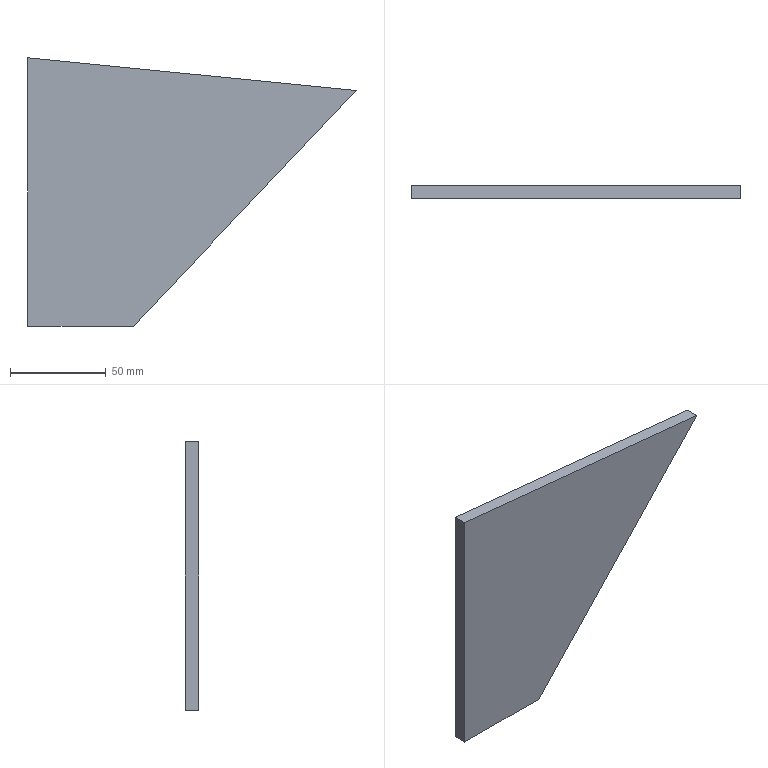Component | NX | TRIANGLE2 | 1 solid | 6 faces | box 171.17 x 7 x 140 mm | volume 107534 mm3 | plane 6
STEP:
#1=CARTESIAN_POINT('',(0.,0.,0.));
#2=DIRECTION('',(0.,0.,1.));
#3=DIRECTION('',(1.,0.,0.));
#4=AXIS2_PLACEMENT_3D('',#1,#2,#3);
#5=CARTESIAN_POINT('',(1430.,1665.,240.032));
#6=VERTEX_POINT('',#5);
#7=CARTESIAN_POINT('',(1546.175,1665.,362.943));
#8=VERTEX_POINT('',#7);
#9=CARTESIAN_POINT('',(1430.,1665.,240.032));
#10=DIRECTION('',(0.6869,0.,0.7267));
#11=VECTOR('',#10,1.);
#12=LINE('',#9,#11);
#13=CARTESIAN_POINT('',(1430.,1658.,240.032));
#14=DIRECTION('',(-0.7267,0.,0.6869));
#15=DIRECTION('',(0.6869,0.,0.7267));
#16=AXIS2_PLACEMENT_3D('',#13,#14,#15);
#17=PLANE('',#16);
#18=CARTESIAN_POINT('',(0.,7.));
#19=DIRECTION('',(1.,0.));
#20=VECTOR('',#19,1.);
#21=LINE('',#18,#20);
#22=(GEOMETRIC_REPRESENTATION_CONTEXT(2)PARAMETRIC_REPRESENTATION_CONTEXT()REPRESENTATION_CONTEXT('',''));
#23=DEFINITIONAL_REPRESENTATION('',(#21),#22);
#24=PCURVE('',#17,#23);
#25=CARTESIAN_POINT('',(1546.175,1665.,362.943));
#26=DIRECTION('',(0.,-1.,0.));
#27=DIRECTION('',(0.,0.,-1.));
#28=AXIS2_PLACEMENT_3D('',#25,#26,#27);
#29=PLANE('',#28);
#30=CARTESIAN_POINT('',(122.911,-116.175));
#31=DIRECTION('',(-0.7267,0.6869));
#32=VECTOR('',#31,1.);
#33=LINE('',#30,#32);
#34=(GEOMETRIC_REPRESENTATION_CONTEXT(2)PARAMETRIC_REPRESENTATION_CONTEXT()REPRESENTATION_CONTEXT('',''));
#35=DEFINITIONAL_REPRESENTATION('',(#33),#34);
#36=PCURVE('',#29,#35);
#37=SURFACE_CURVE('',#12,(#24,#36),.PCURVE_S1.);
#38=EDGE_CURVE('',#6,#8,#37,.T.);
#39=ORIENTED_EDGE('',*,*,#38,.T.);
#40=CARTESIAN_POINT('',(1546.175,1658.,362.943));
#41=VERTEX_POINT('',#40);
#42=CARTESIAN_POINT('',(1546.175,1658.,362.943));
#43=DIRECTION('',(0.,1.,0.));
#44=VECTOR('',#43,1.);
#45=LINE('',#42,#44);
#46=CARTESIAN_POINT('',(169.127,0.));
#47=DIRECTION('',(0.,1.));
#48=VECTOR('',#47,1.);
#49=LINE('',#46,#48);
#50=(GEOMETRIC_REPRESENTATION_CONTEXT(2)PARAMETRIC_REPRESENTATION_CONTEXT()REPRESENTATION_CONTEXT('',''));
#51=DEFINITIONAL_REPRESENTATION('',(#49),#50);
#52=PCURVE('',#17,#51);
#53=CARTESIAN_POINT('',(1546.175,1658.,362.943));
#54=DIRECTION('',(-0.09932,0.,-0.9951));
#55=DIRECTION('',(-0.9951,0.,0.09932));
#56=AXIS2_PLACEMENT_3D('',#53,#54,#55);
#57=PLANE('',#56);
#58=CARTESIAN_POINT('',(0.,0.));
#59=DIRECTION('',(0.,1.));
#60=VECTOR('',#59,1.);
#61=LINE('',#58,#60);
#62=(GEOMETRIC_REPRESENTATION_CONTEXT(2)PARAMETRIC_REPRESENTATION_CONTEXT()REPRESENTATION_CONTEXT('',''));
#63=DEFINITIONAL_REPRESENTATION('',(#61),#62);
#64=PCURVE('',#57,#63);
#65=SURFACE_CURVE('',#45,(#52,#64),.PCURVE_S1.);
#66=EDGE_CURVE('',#41,#8,#65,.T.);
#67=ORIENTED_EDGE('',*,*,#66,.F.);
#68=CARTESIAN_POINT('',(1430.,1658.,240.032));
#69=VERTEX_POINT('',#68);
#70=CARTESIAN_POINT('',(1430.,1658.,240.032));
#71=DIRECTION('',(0.6869,0.,0.7267));
#72=VECTOR('',#71,1.);
#73=LINE('',#70,#72);
#74=CARTESIAN_POINT('',(0.,0.));
#75=DIRECTION('',(1.,0.));
#76=VECTOR('',#75,1.);
#77=LINE('',#74,#76);
#78=(GEOMETRIC_REPRESENTATION_CONTEXT(2)PARAMETRIC_REPRESENTATION_CONTEXT()REPRESENTATION_CONTEXT('',''));
#79=DEFINITIONAL_REPRESENTATION('',(#77),#78);
#80=PCURVE('',#17,#79);
#81=CARTESIAN_POINT('',(1546.175,1658.,362.943));
#82=DIRECTION('',(0.,-1.,0.));
#83=DIRECTION('',(0.,0.,-1.));
#84=AXIS2_PLACEMENT_3D('',#81,#82,#83);
#85=PLANE('',#84);
#86=CARTESIAN_POINT('',(122.911,-116.175));
#87=DIRECTION('',(-0.7267,0.6869));
#88=VECTOR('',#87,1.);
#89=LINE('',#86,#88);
#90=(GEOMETRIC_REPRESENTATION_CONTEXT(2)PARAMETRIC_REPRESENTATION_CONTEXT()REPRESENTATION_CONTEXT('',''));
#91=DEFINITIONAL_REPRESENTATION('',(#89),#90);
#92=PCURVE('',#85,#91);
#93=SURFACE_CURVE('',#73,(#80,#92),.PCURVE_S1.);
#94=EDGE_CURVE('',#69,#41,#93,.T.);
#95=ORIENTED_EDGE('',*,*,#94,.F.);
#96=CARTESIAN_POINT('',(1430.,1658.,240.032));
#97=DIRECTION('',(0.,1.,0.));
#98=VECTOR('',#97,1.);
#99=LINE('',#96,#98);
#100=CARTESIAN_POINT('',(0.,0.));
#101=DIRECTION('',(0.,1.));
#102=VECTOR('',#101,1.);
#103=LINE('',#100,#102);
#104=(GEOMETRIC_REPRESENTATION_CONTEXT(2)PARAMETRIC_REPRESENTATION_CONTEXT()REPRESENTATION_CONTEXT('',''));
#105=DEFINITIONAL_REPRESENTATION('',(#103),#104);
#106=PCURVE('',#17,#105);
#107=CARTESIAN_POINT('',(1375.,1658.,240.032));
#108=DIRECTION('',(0.,0.,1.));
#109=DIRECTION('',(1.,0.,-0.));
#110=AXIS2_PLACEMENT_3D('',#107,#108,#109);
#111=PLANE('',#110);
#112=CARTESIAN_POINT('',(55.,0.));
#113=DIRECTION('',(0.,1.));
#114=VECTOR('',#113,1.);
#115=LINE('',#112,#114);
#116=(GEOMETRIC_REPRESENTATION_CONTEXT(2)PARAMETRIC_REPRESENTATION_CONTEXT()REPRESENTATION_CONTEXT('',''));
#117=DEFINITIONAL_REPRESENTATION('',(#115),#116);
#118=PCURVE('',#111,#117);
#119=SURFACE_CURVE('',#99,(#106,#118),.PCURVE_S1.);
#120=EDGE_CURVE('',#69,#6,#119,.T.);
#121=ORIENTED_EDGE('',*,*,#120,.T.);
#122=EDGE_LOOP('',(#39,#67,#95,#121));
#123=FACE_BOUND('',#122,.T.);
#124=ADVANCED_FACE('',(#123),#17,.F.);
#125=CARTESIAN_POINT('',(1375.,1665.,380.029));
#126=VERTEX_POINT('',#125);
#127=CARTESIAN_POINT('',(1546.175,1665.,362.943));
#128=DIRECTION('',(-0.9951,0.,0.09932));
#129=VECTOR('',#128,1.);
#130=LINE('',#127,#129);
#131=CARTESIAN_POINT('',(0.,7.));
#132=DIRECTION('',(1.,0.));
#133=VECTOR('',#132,1.);
#134=LINE('',#131,#133);
#135=(GEOMETRIC_REPRESENTATION_CONTEXT(2)PARAMETRIC_REPRESENTATION_CONTEXT()REPRESENTATION_CONTEXT('',''));
#136=DEFINITIONAL_REPRESENTATION('',(#134),#135);
#137=PCURVE('',#57,#136);
#138=CARTESIAN_POINT('',(0.,0.));
#139=DIRECTION('',(-0.09932,-0.9951));
#140=VECTOR('',#139,1.);
#141=LINE('',#138,#140);
#142=(GEOMETRIC_REPRESENTATION_CONTEXT(2)PARAMETRIC_REPRESENTATION_CONTEXT()REPRESENTATION_CONTEXT('',''));
#143=DEFINITIONAL_REPRESENTATION('',(#141),#142);
#144=PCURVE('',#29,#143);
#145=SURFACE_CURVE('',#130,(#137,#144),.PCURVE_S1.);
#146=EDGE_CURVE('',#8,#126,#145,.T.);
#147=ORIENTED_EDGE('',*,*,#146,.T.);
#148=CARTESIAN_POINT('',(1375.,1658.,380.029));
#149=VERTEX_POINT('',#148);
#150=CARTESIAN_POINT('',(1375.,1658.,380.029));
#151=DIRECTION('',(0.,1.,0.));
#152=VECTOR('',#151,1.);
#153=LINE('',#150,#152);
#154=CARTESIAN_POINT('',(172.025,0.));
#155=DIRECTION('',(0.,1.));
#156=VECTOR('',#155,1.);
#157=LINE('',#154,#156);
#158=(GEOMETRIC_REPRESENTATION_CONTEXT(2)PARAMETRIC_REPRESENTATION_CONTEXT()REPRESENTATION_CONTEXT('',''));
#159=DEFINITIONAL_REPRESENTATION('',(#157),#158);
#160=PCURVE('',#57,#159);
#161=CARTESIAN_POINT('',(1375.,1658.,380.029));
#162=DIRECTION('',(1.,0.,0.));
#163=DIRECTION('',(0.,0.,-1.));
#164=AXIS2_PLACEMENT_3D('',#161,#162,#163);
#165=PLANE('',#164);
#166=CARTESIAN_POINT('',(0.,0.));
#167=DIRECTION('',(0.,1.));
#168=VECTOR('',#167,1.);
#169=LINE('',#166,#168);
#170=(GEOMETRIC_REPRESENTATION_CONTEXT(2)PARAMETRIC_REPRESENTATION_CONTEXT()REPRESENTATION_CONTEXT('',''));
#171=DEFINITIONAL_REPRESENTATION('',(#169),#170);
#172=PCURVE('',#165,#171);
#173=SURFACE_CURVE('',#153,(#160,#172),.PCURVE_S1.);
#174=EDGE_CURVE('',#149,#126,#173,.T.);
#175=ORIENTED_EDGE('',*,*,#174,.F.);
#176=CARTESIAN_POINT('',(1546.175,1658.,362.943));
#177=DIRECTION('',(-0.9951,0.,0.09932));
#178=VECTOR('',#177,1.);
#179=LINE('',#176,#178);
#180=CARTESIAN_POINT('',(0.,0.));
#181=DIRECTION('',(1.,0.));
#182=VECTOR('',#181,1.);
#183=LINE('',#180,#182);
#184=(GEOMETRIC_REPRESENTATION_CONTEXT(2)PARAMETRIC_REPRESENTATION_CONTEXT()REPRESENTATION_CONTEXT('',''));
#185=DEFINITIONAL_REPRESENTATION('',(#183),#184);
#186=PCURVE('',#57,#185);
#187=CARTESIAN_POINT('',(0.,0.));
#188=DIRECTION('',(-0.09932,-0.9951));
#189=VECTOR('',#188,1.);
#190=LINE('',#187,#189);
#191=(GEOMETRIC_REPRESENTATION_CONTEXT(2)PARAMETRIC_REPRESENTATION_CONTEXT()REPRESENTATION_CONTEXT('',''));
#192=DEFINITIONAL_REPRESENTATION('',(#190),#191);
#193=PCURVE('',#85,#192);
#194=SURFACE_CURVE('',#179,(#186,#193),.PCURVE_S1.);
#195=EDGE_CURVE('',#41,#149,#194,.T.);
#196=ORIENTED_EDGE('',*,*,#195,.F.);
#197=ORIENTED_EDGE('',*,*,#66,.T.);
#198=EDGE_LOOP('',(#147,#175,#196,#197));
#199=FACE_BOUND('',#198,.T.);
#200=ADVANCED_FACE('',(#199),#57,.F.);
#201=CARTESIAN_POINT('',(1375.,1665.,240.032));
#202=VERTEX_POINT('',#201);
#203=CARTESIAN_POINT('',(1375.,1665.,380.029));
#204=DIRECTION('',(0.,0.,-1.));
#205=VECTOR('',#204,1.);
#206=LINE('',#203,#205);
#207=CARTESIAN_POINT('',(0.,7.));
#208=DIRECTION('',(1.,0.));
#209=VECTOR('',#208,1.);
#210=LINE('',#207,#209);
#211=(GEOMETRIC_REPRESENTATION_CONTEXT(2)PARAMETRIC_REPRESENTATION_CONTEXT()REPRESENTATION_CONTEXT('',''));
#212=DEFINITIONAL_REPRESENTATION('',(#210),#211);
#213=PCURVE('',#165,#212);
#214=CARTESIAN_POINT('',(-17.086,-171.175));
#215=DIRECTION('',(1.,0.));
#216=VECTOR('',#215,1.);
#217=LINE('',#214,#216);
#218=(GEOMETRIC_REPRESENTATION_CONTEXT(2)PARAMETRIC_REPRESENTATION_CONTEXT()REPRESENTATION_CONTEXT('',''));
#219=DEFINITIONAL_REPRESENTATION('',(#217),#218);
#220=PCURVE('',#29,#219);
#221=SURFACE_CURVE('',#206,(#213,#220),.PCURVE_S1.);
#222=EDGE_CURVE('',#126,#202,#221,.T.);
#223=ORIENTED_EDGE('',*,*,#222,.T.);
#224=CARTESIAN_POINT('',(1375.,1658.,240.032));
#225=VERTEX_POINT('',#224);
#226=CARTESIAN_POINT('',(1375.,1658.,240.032));
#227=DIRECTION('',(0.,1.,0.));
#228=VECTOR('',#227,1.);
#229=LINE('',#226,#228);
#230=CARTESIAN_POINT('',(139.997,0.));
#231=DIRECTION('',(0.,1.));
#232=VECTOR('',#231,1.);
#233=LINE('',#230,#232);
#234=(GEOMETRIC_REPRESENTATION_CONTEXT(2)PARAMETRIC_REPRESENTATION_CONTEXT()REPRESENTATION_CONTEXT('',''));
#235=DEFINITIONAL_REPRESENTATION('',(#233),#234);
#236=PCURVE('',#165,#235);
#237=CARTESIAN_POINT('',(0.,0.));
#238=DIRECTION('',(0.,1.));
#239=VECTOR('',#238,1.);
#240=LINE('',#237,#239);
#241=(GEOMETRIC_REPRESENTATION_CONTEXT(2)PARAMETRIC_REPRESENTATION_CONTEXT()REPRESENTATION_CONTEXT('',''));
#242=DEFINITIONAL_REPRESENTATION('',(#240),#241);
#243=PCURVE('',#111,#242);
#244=SURFACE_CURVE('',#229,(#236,#243),.PCURVE_S1.);
#245=EDGE_CURVE('',#225,#202,#244,.T.);
#246=ORIENTED_EDGE('',*,*,#245,.F.);
#247=CARTESIAN_POINT('',(1375.,1658.,380.029));
#248=DIRECTION('',(0.,0.,-1.));
#249=VECTOR('',#248,1.);
#250=LINE('',#247,#249);
#251=CARTESIAN_POINT('',(0.,0.));
#252=DIRECTION('',(1.,0.));
#253=VECTOR('',#252,1.);
#254=LINE('',#251,#253);
#255=(GEOMETRIC_REPRESENTATION_CONTEXT(2)PARAMETRIC_REPRESENTATION_CONTEXT()REPRESENTATION_CONTEXT('',''));
#256=DEFINITIONAL_REPRESENTATION('',(#254),#255);
#257=PCURVE('',#165,#256);
#258=CARTESIAN_POINT('',(-17.086,-171.175));
#259=DIRECTION('',(1.,0.));
#260=VECTOR('',#259,1.);
#261=LINE('',#258,#260);
#262=(GEOMETRIC_REPRESENTATION_CONTEXT(2)PARAMETRIC_REPRESENTATION_CONTEXT()REPRESENTATION_CONTEXT('',''));
#263=DEFINITIONAL_REPRESENTATION('',(#261),#262);
#264=PCURVE('',#85,#263);
#265=SURFACE_CURVE('',#250,(#257,#264),.PCURVE_S1.);
#266=EDGE_CURVE('',#149,#225,#265,.T.);
#267=ORIENTED_EDGE('',*,*,#266,.F.);
#268=ORIENTED_EDGE('',*,*,#174,.T.);
#269=EDGE_LOOP('',(#223,#246,#267,#268));
#270=FACE_BOUND('',#269,.T.);
#271=ADVANCED_FACE('',(#270),#165,.F.);
#272=CARTESIAN_POINT('',(1375.,1665.,240.032));
#273=DIRECTION('',(1.,0.,-0.));
#274=VECTOR('',#273,1.);
#275=LINE('',#272,#274);
#276=CARTESIAN_POINT('',(0.,7.));
#277=DIRECTION('',(1.,0.));
#278=VECTOR('',#277,1.);
#279=LINE('',#276,#278);
#280=(GEOMETRIC_REPRESENTATION_CONTEXT(2)PARAMETRIC_REPRESENTATION_CONTEXT()REPRESENTATION_CONTEXT('',''));
#281=DEFINITIONAL_REPRESENTATION('',(#279),#280);
#282=PCURVE('',#111,#281);
#283=CARTESIAN_POINT('',(122.911,-171.175));
#284=DIRECTION('',(0.,1.));
#285=VECTOR('',#284,1.);
#286=LINE('',#283,#285);
#287=(GEOMETRIC_REPRESENTATION_CONTEXT(2)PARAMETRIC_REPRESENTATION_CONTEXT()REPRESENTATION_CONTEXT('',''));
#288=DEFINITIONAL_REPRESENTATION('',(#286),#287);
#289=PCURVE('',#29,#288);
#290=SURFACE_CURVE('',#275,(#282,#289),.PCURVE_S1.);
#291=EDGE_CURVE('',#202,#6,#290,.T.);
#292=ORIENTED_EDGE('',*,*,#291,.T.);
#293=ORIENTED_EDGE('',*,*,#120,.F.);
#294=CARTESIAN_POINT('',(1375.,1658.,240.032));
#295=DIRECTION('',(1.,0.,-0.));
#296=VECTOR('',#295,1.);
#297=LINE('',#294,#296);
#298=CARTESIAN_POINT('',(0.,0.));
#299=DIRECTION('',(1.,0.));
#300=VECTOR('',#299,1.);
#301=LINE('',#298,#300);
#302=(GEOMETRIC_REPRESENTATION_CONTEXT(2)PARAMETRIC_REPRESENTATION_CONTEXT()REPRESENTATION_CONTEXT('',''));
#303=DEFINITIONAL_REPRESENTATION('',(#301),#302);
#304=PCURVE('',#111,#303);
#305=CARTESIAN_POINT('',(122.911,-171.175));
#306=DIRECTION('',(0.,1.));
#307=VECTOR('',#306,1.);
#308=LINE('',#305,#307);
#309=(GEOMETRIC_REPRESENTATION_CONTEXT(2)PARAMETRIC_REPRESENTATION_CONTEXT()REPRESENTATION_CONTEXT('',''));
#310=DEFINITIONAL_REPRESENTATION('',(#308),#309);
#311=PCURVE('',#85,#310);
#312=SURFACE_CURVE('',#297,(#304,#311),.PCURVE_S1.);
#313=EDGE_CURVE('',#225,#69,#312,.T.);
#314=ORIENTED_EDGE('',*,*,#313,.F.);
#315=ORIENTED_EDGE('',*,*,#245,.T.);
#316=EDGE_LOOP('',(#292,#293,#314,#315));
#317=FACE_BOUND('',#316,.T.);
#318=ADVANCED_FACE('',(#317),#111,.F.);
#319=ORIENTED_EDGE('',*,*,#94,.T.);
#320=ORIENTED_EDGE('',*,*,#195,.T.);
#321=ORIENTED_EDGE('',*,*,#266,.T.);
#322=ORIENTED_EDGE('',*,*,#313,.T.);
#323=EDGE_LOOP('',(#319,#320,#321,#322));
#324=FACE_BOUND('',#323,.T.);
#325=ADVANCED_FACE('',(#324),#85,.T.);
#326=ORIENTED_EDGE('',*,*,#38,.F.);
#327=ORIENTED_EDGE('',*,*,#291,.F.);
#328=ORIENTED_EDGE('',*,*,#222,.F.);
#329=ORIENTED_EDGE('',*,*,#146,.F.);
#330=EDGE_LOOP('',(#326,#327,#328,#329));
#331=FACE_BOUND('',#330,.T.);
#332=ADVANCED_FACE('',(#331),#29,.F.);
#333=CLOSED_SHELL('',(#124,#200,#271,#318,#325,#332));
#334=MANIFOLD_SOLID_BREP('',#333);
#335=(LENGTH_UNIT()NAMED_UNIT(*)SI_UNIT(.MILLI.,.METRE.));
#336=UNCERTAINTY_MEASURE_WITH_UNIT(LENGTH_MEASURE(0.0000001),#335,'','');
#337=(NAMED_UNIT(*)PLANE_ANGLE_UNIT()SI_UNIT($,.RADIAN.));
#338=(NAMED_UNIT(*)SI_UNIT($,.STERADIAN.)SOLID_ANGLE_UNIT());
#339=(GEOMETRIC_REPRESENTATION_CONTEXT(3)GLOBAL_UNCERTAINTY_ASSIGNED_CONTEXT((#336))GLOBAL_UNIT_ASSIGNED_CONTEXT((#335,#337,#338))REPRESENTATION_CONTEXT('',''));
#340=ADVANCED_BREP_SHAPE_REPRESENTATION('',(#4,#334),#339);